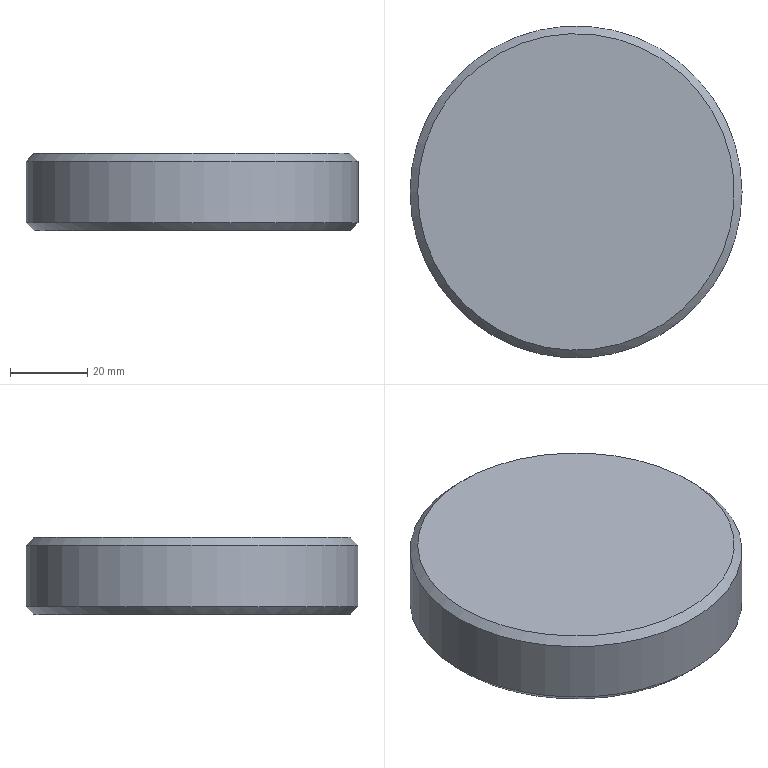Component | NX | CH3404_19_3-1 | 1 solid | 9 faces | box 86 x 86 x 20 mm | volume 33415 mm3 | plane 4 | cylinder 3 | cone 2 | commonest cylinder face diameters 86 x1 80 x1 82 x1
STEP:
#1=CARTESIAN_POINT('',(0.,0.,0.));
#2=DIRECTION('',(0.,0.,1.));
#3=DIRECTION('',(1.,0.,0.));
#4=AXIS2_PLACEMENT_3D('',#1,#2,#3);
#5=CARTESIAN_POINT('',(43.,0.,91.55));
#6=VERTEX_POINT('',#5);
#7=CARTESIAN_POINT('',(-43.,0.,91.55));
#8=VERTEX_POINT('',#7);
#9=CARTESIAN_POINT('',(-0.,0.,91.55));
#10=DIRECTION('',(0.,0.,1.));
#11=DIRECTION('',(1.,0.,0.));
#12=AXIS2_PLACEMENT_3D('',#9,#10,#11);
#13=CIRCLE('',#12,43.);
#14=CARTESIAN_POINT('',(-0.,0.,89.55));
#15=DIRECTION('',(0.,0.,-1.));
#16=DIRECTION('',(-1.,0.,0.));
#17=AXIS2_PLACEMENT_3D('',#14,#15,#16);
#18=CYLINDRICAL_SURFACE('',#17,43.);
#19=CARTESIAN_POINT('',(3.142,-2.));
#20=DIRECTION('',(-1.,0.));
#21=VECTOR('',#20,1.);
#22=LINE('',#19,#21);
#23=(GEOMETRIC_REPRESENTATION_CONTEXT(2)PARAMETRIC_REPRESENTATION_CONTEXT()REPRESENTATION_CONTEXT('',''));
#24=DEFINITIONAL_REPRESENTATION('',(#22),#23);
#25=PCURVE('',#18,#24);
#26=CARTESIAN_POINT('',(-0.,0.,89.55));
#27=DIRECTION('',(0.,0.,1.));
#28=DIRECTION('',(1.,0.,0.));
#29=AXIS2_PLACEMENT_3D('',#26,#27,#28);
#30=CONICAL_SURFACE('',#29,41.,0.7854);
#31=CARTESIAN_POINT('',(0.,2.));
#32=DIRECTION('',(1.,0.));
#33=VECTOR('',#32,1.);
#34=LINE('',#31,#33);
#35=(GEOMETRIC_REPRESENTATION_CONTEXT(2)PARAMETRIC_REPRESENTATION_CONTEXT()REPRESENTATION_CONTEXT('',''));
#36=DEFINITIONAL_REPRESENTATION('',(#34),#35);
#37=PCURVE('',#30,#36);
#38=SURFACE_CURVE('',#13,(#25,#37),.PCURVE_S1.);
#39=EDGE_CURVE('',#6,#8,#38,.T.);
#40=ORIENTED_EDGE('',*,*,#39,.T.);
#41=CARTESIAN_POINT('',(-43.,0.,107.55));
#42=VERTEX_POINT('',#41);
#43=CARTESIAN_POINT('',(-43.,-0.,107.55));
#44=CARTESIAN_POINT('',(-43.,-0.,91.55));
#45=B_SPLINE_CURVE_WITH_KNOTS('',1,(#43,#44),.UNSPECIFIED.,.F.,.F.,(2,2),(-18.,-2.),.PIECEWISE_BEZIER_KNOTS.);
#46=CARTESIAN_POINT('',(0.,0.));
#47=DIRECTION('',(0.,1.));
#48=VECTOR('',#47,1.);
#49=LINE('',#46,#48);
#50=(GEOMETRIC_REPRESENTATION_CONTEXT(2)PARAMETRIC_REPRESENTATION_CONTEXT()REPRESENTATION_CONTEXT('',''));
#51=DEFINITIONAL_REPRESENTATION('',(#49),#50);
#52=PCURVE('',#18,#51);
#53=CARTESIAN_POINT('',(6.283,0.));
#54=DIRECTION('',(0.,1.));
#55=VECTOR('',#54,1.);
#56=LINE('',#53,#55);
#57=(GEOMETRIC_REPRESENTATION_CONTEXT(2)PARAMETRIC_REPRESENTATION_CONTEXT()REPRESENTATION_CONTEXT('',''));
#58=DEFINITIONAL_REPRESENTATION('',(#56),#57);
#59=PCURVE('',#18,#58);
#60=SEAM_CURVE('',#45,(#52,#59),.PCURVE_S1.);
#61=EDGE_CURVE('',#42,#8,#60,.T.);
#62=ORIENTED_EDGE('',*,*,#61,.F.);
#63=CARTESIAN_POINT('',(-0.,0.,107.55));
#64=DIRECTION('',(0.,0.,-1.));
#65=DIRECTION('',(-1.,0.,0.));
#66=AXIS2_PLACEMENT_3D('',#63,#64,#65);
#67=CIRCLE('',#66,43.);
#68=CARTESIAN_POINT('',(0.,-18.));
#69=DIRECTION('',(1.,0.));
#70=VECTOR('',#69,1.);
#71=LINE('',#68,#70);
#72=(GEOMETRIC_REPRESENTATION_CONTEXT(2)PARAMETRIC_REPRESENTATION_CONTEXT()REPRESENTATION_CONTEXT('',''));
#73=DEFINITIONAL_REPRESENTATION('',(#71),#72);
#74=PCURVE('',#18,#73);
#75=CARTESIAN_POINT('',(-0.,0.,107.55));
#76=DIRECTION('',(0.,0.,-1.));
#77=DIRECTION('',(-1.,0.,0.));
#78=AXIS2_PLACEMENT_3D('',#75,#76,#77);
#79=CONICAL_SURFACE('',#78,43.,0.7854);
#80=CARTESIAN_POINT('',(0.,0.));
#81=DIRECTION('',(1.,0.));
#82=VECTOR('',#81,1.);
#83=LINE('',#80,#82);
#84=(GEOMETRIC_REPRESENTATION_CONTEXT(2)PARAMETRIC_REPRESENTATION_CONTEXT()REPRESENTATION_CONTEXT('',''));
#85=DEFINITIONAL_REPRESENTATION('',(#83),#84);
#86=PCURVE('',#79,#85);
#87=SURFACE_CURVE('',#67,(#74,#86),.PCURVE_S1.);
#88=EDGE_CURVE('',#42,#42,#87,.T.);
#89=ORIENTED_EDGE('',*,*,#88,.T.);
#90=ORIENTED_EDGE('',*,*,#61,.T.);
#91=CARTESIAN_POINT('',(-0.,0.,91.55));
#92=DIRECTION('',(0.,0.,1.));
#93=DIRECTION('',(1.,0.,0.));
#94=AXIS2_PLACEMENT_3D('',#91,#92,#93);
#95=CIRCLE('',#94,43.);
#96=CARTESIAN_POINT('',(9.425,-2.));
#97=DIRECTION('',(-1.,0.));
#98=VECTOR('',#97,1.);
#99=LINE('',#96,#98);
#100=(GEOMETRIC_REPRESENTATION_CONTEXT(2)PARAMETRIC_REPRESENTATION_CONTEXT()REPRESENTATION_CONTEXT('',''));
#101=DEFINITIONAL_REPRESENTATION('',(#99),#100);
#102=PCURVE('',#18,#101);
#103=CARTESIAN_POINT('',(0.,2.));
#104=DIRECTION('',(1.,0.));
#105=VECTOR('',#104,1.);
#106=LINE('',#103,#105);
#107=(GEOMETRIC_REPRESENTATION_CONTEXT(2)PARAMETRIC_REPRESENTATION_CONTEXT()REPRESENTATION_CONTEXT('',''));
#108=DEFINITIONAL_REPRESENTATION('',(#106),#107);
#109=PCURVE('',#30,#108);
#110=SURFACE_CURVE('',#95,(#102,#109),.PCURVE_S1.);
#111=EDGE_CURVE('',#8,#6,#110,.T.);
#112=ORIENTED_EDGE('',*,*,#111,.T.);
#113=EDGE_LOOP('',(#40,#62,#89,#90,#112));
#114=FACE_BOUND('',#113,.T.);
#115=ADVANCED_FACE('',(#114),#18,.T.);
#116=CARTESIAN_POINT('',(41.,0.,89.55));
#117=VERTEX_POINT('',#116);
#118=CARTESIAN_POINT('',(-0.,0.,89.55));
#119=DIRECTION('',(0.,0.,-1.));
#120=DIRECTION('',(1.,0.,0.));
#121=AXIS2_PLACEMENT_3D('',#118,#119,#120);
#122=CIRCLE('',#121,41.);
#123=CARTESIAN_POINT('',(-0.,-43.,89.55));
#124=DIRECTION('',(0.,0.,1.));
#125=DIRECTION('',(1.,0.,0.));
#126=AXIS2_PLACEMENT_3D('',#123,#124,#125);
#127=PLANE('',#126);
#128=CARTESIAN_POINT('',(41.,43.));
#129=CARTESIAN_POINT('',(41.,-28.014));
#130=CARTESIAN_POINT('',(-20.5,7.493));
#131=CARTESIAN_POINT('',(-82.,43.));
#132=CARTESIAN_POINT('',(-20.5,78.507));
#133=CARTESIAN_POINT('',(41.,114.014));
#134=CARTESIAN_POINT('',(41.,43.));
#135=(BOUNDED_CURVE()B_SPLINE_CURVE(2,(#128,#129,#130,#131,#132,#133,#134),.UNSPECIFIED.,.T.,.F.)B_SPLINE_CURVE_WITH_KNOTS((1,2,2,2,2,1),(-2.094,0.,2.094,4.189,6.283,8.378),.UNSPECIFIED.)CURVE()GEOMETRIC_REPRESENTATION_ITEM()RATIONAL_B_SPLINE_CURVE((1.,0.5,1.,0.5,1.,0.5,1.))REPRESENTATION_ITEM(''));
#136=(GEOMETRIC_REPRESENTATION_CONTEXT(2)PARAMETRIC_REPRESENTATION_CONTEXT()REPRESENTATION_CONTEXT('',''));
#137=DEFINITIONAL_REPRESENTATION('',(#135),#136);
#138=PCURVE('',#127,#137);
#139=CARTESIAN_POINT('',(6.283,0.));
#140=DIRECTION('',(-1.,0.));
#141=VECTOR('',#140,1.);
#142=LINE('',#139,#141);
#143=(GEOMETRIC_REPRESENTATION_CONTEXT(2)PARAMETRIC_REPRESENTATION_CONTEXT()REPRESENTATION_CONTEXT('',''));
#144=DEFINITIONAL_REPRESENTATION('',(#142),#143);
#145=PCURVE('',#30,#144);
#146=SURFACE_CURVE('',#122,(#138,#145),.PCURVE_S1.);
#147=EDGE_CURVE('',#117,#117,#146,.T.);
#148=ORIENTED_EDGE('',*,*,#147,.T.);
#149=EDGE_LOOP('',(#148));
#150=FACE_BOUND('',#149,.T.);
#151=CARTESIAN_POINT('',(-40.,0.,89.55));
#152=VERTEX_POINT('',#151);
#153=CARTESIAN_POINT('',(-0.,0.,89.55));
#154=DIRECTION('',(0.,0.,-1.));
#155=DIRECTION('',(-1.,0.,0.));
#156=AXIS2_PLACEMENT_3D('',#153,#154,#155);
#157=CIRCLE('',#156,40.);
#158=CARTESIAN_POINT('',(-40.,43.));
#159=CARTESIAN_POINT('',(-40.,112.282));
#160=CARTESIAN_POINT('',(20.,77.641));
#161=CARTESIAN_POINT('',(80.,43.));
#162=CARTESIAN_POINT('',(20.,8.359));
#163=CARTESIAN_POINT('',(-40.,-26.282));
#164=CARTESIAN_POINT('',(-40.,43.));
#165=(BOUNDED_CURVE()B_SPLINE_CURVE(2,(#158,#159,#160,#161,#162,#163,#164),.UNSPECIFIED.,.T.,.F.)B_SPLINE_CURVE_WITH_KNOTS((1,2,2,2,2,1),(-2.094,0.,2.094,4.189,6.283,8.378),.UNSPECIFIED.)CURVE()GEOMETRIC_REPRESENTATION_ITEM()RATIONAL_B_SPLINE_CURVE((1.,0.5,1.,0.5,1.,0.5,1.))REPRESENTATION_ITEM(''));
#166=(GEOMETRIC_REPRESENTATION_CONTEXT(2)PARAMETRIC_REPRESENTATION_CONTEXT()REPRESENTATION_CONTEXT('',''));
#167=DEFINITIONAL_REPRESENTATION('',(#165),#166);
#168=PCURVE('',#127,#167);
#169=CARTESIAN_POINT('',(-0.,0.,89.55));
#170=DIRECTION('',(0.,0.,-1.));
#171=DIRECTION('',(-1.,0.,0.));
#172=AXIS2_PLACEMENT_3D('',#169,#170,#171);
#173=CYLINDRICAL_SURFACE('',#172,40.);
#174=CARTESIAN_POINT('',(0.,0.));
#175=DIRECTION('',(1.,0.));
#176=VECTOR('',#175,1.);
#177=LINE('',#174,#176);
#178=(GEOMETRIC_REPRESENTATION_CONTEXT(2)PARAMETRIC_REPRESENTATION_CONTEXT()REPRESENTATION_CONTEXT('',''));
#179=DEFINITIONAL_REPRESENTATION('',(#177),#178);
#180=PCURVE('',#173,#179);
#181=SURFACE_CURVE('',#157,(#168,#180),.PCURVE_S1.);
#182=EDGE_CURVE('',#152,#152,#181,.T.);
#183=ORIENTED_EDGE('',*,*,#182,.F.);
#184=EDGE_LOOP('',(#183));
#185=FACE_BOUND('',#184,.T.);
#186=ADVANCED_FACE('',(#150,#185),#127,.F.);
#187=CARTESIAN_POINT('',(-40.,0.,100.55));
#188=VERTEX_POINT('',#187);
#189=CARTESIAN_POINT('',(-0.,0.,100.55));
#190=DIRECTION('',(0.,0.,-1.));
#191=DIRECTION('',(-1.,0.,0.));
#192=AXIS2_PLACEMENT_3D('',#189,#190,#191);
#193=CIRCLE('',#192,40.);
#194=CARTESIAN_POINT('',(0.,-11.));
#195=DIRECTION('',(1.,0.));
#196=VECTOR('',#195,1.);
#197=LINE('',#194,#196);
#198=(GEOMETRIC_REPRESENTATION_CONTEXT(2)PARAMETRIC_REPRESENTATION_CONTEXT()REPRESENTATION_CONTEXT('',''));
#199=DEFINITIONAL_REPRESENTATION('',(#197),#198);
#200=PCURVE('',#173,#199);
#201=CARTESIAN_POINT('',(-0.,-40.,100.55));
#202=DIRECTION('',(0.,0.,-1.));
#203=DIRECTION('',(-1.,0.,0.));
#204=AXIS2_PLACEMENT_3D('',#201,#202,#203);
#205=PLANE('',#204);
#206=CARTESIAN_POINT('',(0.,40.));
#207=DIRECTION('',(1.,0.));
#208=AXIS2_PLACEMENT_2D('',#206,#207);
#209=CIRCLE('',#208,40.);
#210=(GEOMETRIC_REPRESENTATION_CONTEXT(2)PARAMETRIC_REPRESENTATION_CONTEXT()REPRESENTATION_CONTEXT('',''));
#211=DEFINITIONAL_REPRESENTATION('',(#209),#210);
#212=PCURVE('',#205,#211);
#213=SURFACE_CURVE('',#193,(#200,#212),.PCURVE_S1.);
#214=EDGE_CURVE('',#188,#188,#213,.T.);
#215=ORIENTED_EDGE('',*,*,#214,.T.);
#216=CARTESIAN_POINT('',(-40.,0.,100.55));
#217=CARTESIAN_POINT('',(-40.,0.,89.55));
#218=B_SPLINE_CURVE_WITH_KNOTS('',1,(#216,#217),.UNSPECIFIED.,.F.,.F.,(2,2),(-11.,0.),.PIECEWISE_BEZIER_KNOTS.);
#219=CARTESIAN_POINT('',(6.283,0.));
#220=DIRECTION('',(0.,1.));
#221=VECTOR('',#220,1.);
#222=LINE('',#219,#221);
#223=(GEOMETRIC_REPRESENTATION_CONTEXT(2)PARAMETRIC_REPRESENTATION_CONTEXT()REPRESENTATION_CONTEXT('',''));
#224=DEFINITIONAL_REPRESENTATION('',(#222),#223);
#225=PCURVE('',#173,#224);
#226=CARTESIAN_POINT('',(0.,0.));
#227=DIRECTION('',(0.,1.));
#228=VECTOR('',#227,1.);
#229=LINE('',#226,#228);
#230=(GEOMETRIC_REPRESENTATION_CONTEXT(2)PARAMETRIC_REPRESENTATION_CONTEXT()REPRESENTATION_CONTEXT('',''));
#231=DEFINITIONAL_REPRESENTATION('',(#229),#230);
#232=PCURVE('',#173,#231);
#233=SEAM_CURVE('',#218,(#225,#232),.PCURVE_S1.);
#234=EDGE_CURVE('',#188,#152,#233,.T.);
#235=ORIENTED_EDGE('',*,*,#234,.T.);
#236=ORIENTED_EDGE('',*,*,#182,.F.);
#237=ORIENTED_EDGE('',*,*,#234,.F.);
#238=EDGE_LOOP('',(#215,#235,#236,#237));
#239=FACE_BOUND('',#238,.F.);
#240=ADVANCED_FACE('',(#239),#173,.F.);
#241=CARTESIAN_POINT('',(-41.,0.,100.55));
#242=VERTEX_POINT('',#241);
#243=CARTESIAN_POINT('',(-0.,0.,100.55));
#244=DIRECTION('',(0.,0.,-1.));
#245=DIRECTION('',(-1.,0.,0.));
#246=AXIS2_PLACEMENT_3D('',#243,#244,#245);
#247=CIRCLE('',#246,41.);
#248=CARTESIAN_POINT('',(0.,40.));
#249=DIRECTION('',(1.,0.));
#250=AXIS2_PLACEMENT_2D('',#248,#249);
#251=CIRCLE('',#250,41.);
#252=(GEOMETRIC_REPRESENTATION_CONTEXT(2)PARAMETRIC_REPRESENTATION_CONTEXT()REPRESENTATION_CONTEXT('',''));
#253=DEFINITIONAL_REPRESENTATION('',(#251),#252);
#254=PCURVE('',#205,#253);
#255=CARTESIAN_POINT('',(-0.,0.,89.55));
#256=DIRECTION('',(0.,0.,-1.));
#257=DIRECTION('',(-1.,0.,0.));
#258=AXIS2_PLACEMENT_3D('',#255,#256,#257);
#259=CYLINDRICAL_SURFACE('',#258,41.);
#260=CARTESIAN_POINT('',(0.,-11.));
#261=DIRECTION('',(1.,0.));
#262=VECTOR('',#261,1.);
#263=LINE('',#260,#262);
#264=(GEOMETRIC_REPRESENTATION_CONTEXT(2)PARAMETRIC_REPRESENTATION_CONTEXT()REPRESENTATION_CONTEXT('',''));
#265=DEFINITIONAL_REPRESENTATION('',(#263),#264);
#266=PCURVE('',#259,#265);
#267=SURFACE_CURVE('',#247,(#254,#266),.PCURVE_S1.);
#268=EDGE_CURVE('',#242,#242,#267,.T.);
#269=ORIENTED_EDGE('',*,*,#268,.F.);
#270=EDGE_LOOP('',(#269));
#271=FACE_BOUND('',#270,.T.);
#272=ORIENTED_EDGE('',*,*,#214,.T.);
#273=EDGE_LOOP('',(#272));
#274=FACE_BOUND('',#273,.T.);
#275=ADVANCED_FACE('',(#271,#274),#205,.F.);
#276=CARTESIAN_POINT('',(-41.,0.,105.55));
#277=VERTEX_POINT('',#276);
#278=CARTESIAN_POINT('',(-0.,0.,105.55));
#279=DIRECTION('',(0.,0.,-1.));
#280=DIRECTION('',(-1.,0.,0.));
#281=AXIS2_PLACEMENT_3D('',#278,#279,#280);
#282=CIRCLE('',#281,41.);
#283=CARTESIAN_POINT('',(0.,-16.));
#284=DIRECTION('',(1.,0.));
#285=VECTOR('',#284,1.);
#286=LINE('',#283,#285);
#287=(GEOMETRIC_REPRESENTATION_CONTEXT(2)PARAMETRIC_REPRESENTATION_CONTEXT()REPRESENTATION_CONTEXT('',''));
#288=DEFINITIONAL_REPRESENTATION('',(#286),#287);
#289=PCURVE('',#259,#288);
#290=CARTESIAN_POINT('',(-0.,-41.,105.55));
#291=DIRECTION('',(0.,0.,1.));
#292=DIRECTION('',(1.,0.,0.));
#293=AXIS2_PLACEMENT_3D('',#290,#291,#292);
#294=PLANE('',#293);
#295=CARTESIAN_POINT('',(-41.,41.));
#296=CARTESIAN_POINT('',(-41.,112.014));
#297=CARTESIAN_POINT('',(20.5,76.507));
#298=CARTESIAN_POINT('',(82.,41.));
#299=CARTESIAN_POINT('',(20.5,5.493));
#300=CARTESIAN_POINT('',(-41.,-30.014));
#301=CARTESIAN_POINT('',(-41.,41.));
#302=(BOUNDED_CURVE()B_SPLINE_CURVE(2,(#295,#296,#297,#298,#299,#300,#301),.UNSPECIFIED.,.T.,.F.)B_SPLINE_CURVE_WITH_KNOTS((1,2,2,2,2,1),(-2.094,0.,2.094,4.189,6.283,8.378),.UNSPECIFIED.)CURVE()GEOMETRIC_REPRESENTATION_ITEM()RATIONAL_B_SPLINE_CURVE((1.,0.5,1.,0.5,1.,0.5,1.))REPRESENTATION_ITEM(''));
#303=(GEOMETRIC_REPRESENTATION_CONTEXT(2)PARAMETRIC_REPRESENTATION_CONTEXT()REPRESENTATION_CONTEXT('',''));
#304=DEFINITIONAL_REPRESENTATION('',(#302),#303);
#305=PCURVE('',#294,#304);
#306=SURFACE_CURVE('',#282,(#289,#305),.PCURVE_S1.);
#307=EDGE_CURVE('',#277,#277,#306,.T.);
#308=ORIENTED_EDGE('',*,*,#307,.T.);
#309=CARTESIAN_POINT('',(-41.,0.,105.55));
#310=CARTESIAN_POINT('',(-41.,0.,100.55));
#311=B_SPLINE_CURVE_WITH_KNOTS('',1,(#309,#310),.UNSPECIFIED.,.F.,.F.,(2,2),(-16.,-11.),.PIECEWISE_BEZIER_KNOTS.);
#312=CARTESIAN_POINT('',(6.283,0.));
#313=DIRECTION('',(0.,1.));
#314=VECTOR('',#313,1.);
#315=LINE('',#312,#314);
#316=(GEOMETRIC_REPRESENTATION_CONTEXT(2)PARAMETRIC_REPRESENTATION_CONTEXT()REPRESENTATION_CONTEXT('',''));
#317=DEFINITIONAL_REPRESENTATION('',(#315),#316);
#318=PCURVE('',#259,#317);
#319=CARTESIAN_POINT('',(0.,0.));
#320=DIRECTION('',(0.,1.));
#321=VECTOR('',#320,1.);
#322=LINE('',#319,#321);
#323=(GEOMETRIC_REPRESENTATION_CONTEXT(2)PARAMETRIC_REPRESENTATION_CONTEXT()REPRESENTATION_CONTEXT('',''));
#324=DEFINITIONAL_REPRESENTATION('',(#322),#323);
#325=PCURVE('',#259,#324);
#326=SEAM_CURVE('',#311,(#318,#325),.PCURVE_S1.);
#327=EDGE_CURVE('',#277,#242,#326,.T.);
#328=ORIENTED_EDGE('',*,*,#327,.T.);
#329=ORIENTED_EDGE('',*,*,#268,.F.);
#330=ORIENTED_EDGE('',*,*,#327,.F.);
#331=EDGE_LOOP('',(#308,#328,#329,#330));
#332=FACE_BOUND('',#331,.F.);
#333=ADVANCED_FACE('',(#332),#259,.F.);
#334=ORIENTED_EDGE('',*,*,#307,.T.);
#335=EDGE_LOOP('',(#334));
#336=FACE_BOUND('',#335,.T.);
#337=ADVANCED_FACE('',(#336),#294,.F.);
#338=CARTESIAN_POINT('',(-41.,0.,109.55));
#339=VERTEX_POINT('',#338);
#340=CARTESIAN_POINT('',(-0.,0.,109.55));
#341=DIRECTION('',(0.,0.,1.));
#342=DIRECTION('',(-1.,0.,0.));
#343=AXIS2_PLACEMENT_3D('',#340,#341,#342);
#344=CIRCLE('',#343,41.);
#345=CARTESIAN_POINT('',(-0.,0.,109.55));
#346=DIRECTION('',(0.,0.,-1.));
#347=DIRECTION('',(-1.,0.,0.));
#348=AXIS2_PLACEMENT_3D('',#345,#346,#347);
#349=PLANE('',#348);
#350=CARTESIAN_POINT('',(41.,0.));
#351=CARTESIAN_POINT('',(41.,-71.014));
#352=CARTESIAN_POINT('',(-20.5,-35.507));
#353=CARTESIAN_POINT('',(-82.,-0.));
#354=CARTESIAN_POINT('',(-20.5,35.507));
#355=CARTESIAN_POINT('',(41.,71.014));
#356=CARTESIAN_POINT('',(41.,0.));
#357=(BOUNDED_CURVE()B_SPLINE_CURVE(2,(#350,#351,#352,#353,#354,#355,#356),.UNSPECIFIED.,.T.,.F.)B_SPLINE_CURVE_WITH_KNOTS((1,2,2,2,2,1),(-2.094,0.,2.094,4.189,6.283,8.378),.UNSPECIFIED.)CURVE()GEOMETRIC_REPRESENTATION_ITEM()RATIONAL_B_SPLINE_CURVE((1.,0.5,1.,0.5,1.,0.5,1.))REPRESENTATION_ITEM(''));
#358=(GEOMETRIC_REPRESENTATION_CONTEXT(2)PARAMETRIC_REPRESENTATION_CONTEXT()REPRESENTATION_CONTEXT('',''));
#359=DEFINITIONAL_REPRESENTATION('',(#357),#358);
#360=PCURVE('',#349,#359);
#361=CARTESIAN_POINT('',(6.283,-2.));
#362=DIRECTION('',(-1.,0.));
#363=VECTOR('',#362,1.);
#364=LINE('',#361,#363);
#365=(GEOMETRIC_REPRESENTATION_CONTEXT(2)PARAMETRIC_REPRESENTATION_CONTEXT()REPRESENTATION_CONTEXT('',''));
#366=DEFINITIONAL_REPRESENTATION('',(#364),#365);
#367=PCURVE('',#79,#366);
#368=SURFACE_CURVE('',#344,(#360,#367),.PCURVE_S1.);
#369=EDGE_CURVE('',#339,#339,#368,.T.);
#370=ORIENTED_EDGE('',*,*,#369,.T.);
#371=EDGE_LOOP('',(#370));
#372=FACE_BOUND('',#371,.T.);
#373=ADVANCED_FACE('',(#372),#349,.F.);
#374=ORIENTED_EDGE('',*,*,#39,.F.);
#375=CARTESIAN_POINT('',(41.,-0.,89.55));
#376=CARTESIAN_POINT('',(43.,-0.,91.55));
#377=B_SPLINE_CURVE_WITH_KNOTS('',1,(#375,#376),.UNSPECIFIED.,.F.,.F.,(2,2),(0.,2.828),.PIECEWISE_BEZIER_KNOTS.);
#378=CARTESIAN_POINT('',(0.,0.));
#379=DIRECTION('',(0.,1.));
#380=VECTOR('',#379,1.);
#381=LINE('',#378,#380);
#382=(GEOMETRIC_REPRESENTATION_CONTEXT(2)PARAMETRIC_REPRESENTATION_CONTEXT()REPRESENTATION_CONTEXT('',''));
#383=DEFINITIONAL_REPRESENTATION('',(#381),#382);
#384=PCURVE('',#30,#383);
#385=CARTESIAN_POINT('',(6.283,0.));
#386=DIRECTION('',(0.,1.));
#387=VECTOR('',#386,1.);
#388=LINE('',#385,#387);
#389=(GEOMETRIC_REPRESENTATION_CONTEXT(2)PARAMETRIC_REPRESENTATION_CONTEXT()REPRESENTATION_CONTEXT('',''));
#390=DEFINITIONAL_REPRESENTATION('',(#388),#389);
#391=PCURVE('',#30,#390);
#392=SEAM_CURVE('',#377,(#384,#391),.PCURVE_S1.);
#393=EDGE_CURVE('',#117,#6,#392,.T.);
#394=ORIENTED_EDGE('',*,*,#393,.F.);
#395=ORIENTED_EDGE('',*,*,#147,.F.);
#396=ORIENTED_EDGE('',*,*,#393,.T.);
#397=ORIENTED_EDGE('',*,*,#111,.F.);
#398=EDGE_LOOP('',(#374,#394,#395,#396,#397));
#399=FACE_BOUND('',#398,.T.);
#400=ADVANCED_FACE('',(#399),#30,.T.);
#401=ORIENTED_EDGE('',*,*,#369,.F.);
#402=CARTESIAN_POINT('',(-41.,0.,109.55));
#403=CARTESIAN_POINT('',(-43.,0.,107.55));
#404=B_SPLINE_CURVE_WITH_KNOTS('',1,(#402,#403),.UNSPECIFIED.,.F.,.F.,(2,2),(-2.828,0.),.PIECEWISE_BEZIER_KNOTS.);
#405=CARTESIAN_POINT('',(6.283,0.));
#406=DIRECTION('',(0.,1.));
#407=VECTOR('',#406,1.);
#408=LINE('',#405,#407);
#409=(GEOMETRIC_REPRESENTATION_CONTEXT(2)PARAMETRIC_REPRESENTATION_CONTEXT()REPRESENTATION_CONTEXT('',''));
#410=DEFINITIONAL_REPRESENTATION('',(#408),#409);
#411=PCURVE('',#79,#410);
#412=CARTESIAN_POINT('',(0.,0.));
#413=DIRECTION('',(0.,1.));
#414=VECTOR('',#413,1.);
#415=LINE('',#412,#414);
#416=(GEOMETRIC_REPRESENTATION_CONTEXT(2)PARAMETRIC_REPRESENTATION_CONTEXT()REPRESENTATION_CONTEXT('',''));
#417=DEFINITIONAL_REPRESENTATION('',(#415),#416);
#418=PCURVE('',#79,#417);
#419=SEAM_CURVE('',#404,(#411,#418),.PCURVE_S1.);
#420=EDGE_CURVE('',#339,#42,#419,.T.);
#421=ORIENTED_EDGE('',*,*,#420,.T.);
#422=ORIENTED_EDGE('',*,*,#88,.F.);
#423=ORIENTED_EDGE('',*,*,#420,.F.);
#424=EDGE_LOOP('',(#401,#421,#422,#423));
#425=FACE_BOUND('',#424,.T.);
#426=ADVANCED_FACE('',(#425),#79,.T.);
#427=CLOSED_SHELL('',(#115,#186,#240,#275,#333,#337,#373,#400,#426));
#428=MANIFOLD_SOLID_BREP('',#427);
#429=(LENGTH_UNIT()NAMED_UNIT(*)SI_UNIT(.MILLI.,.METRE.));
#430=UNCERTAINTY_MEASURE_WITH_UNIT(LENGTH_MEASURE(0.00001),#429,'','');
#431=(NAMED_UNIT(*)PLANE_ANGLE_UNIT()SI_UNIT($,.RADIAN.));
#432=(NAMED_UNIT(*)SI_UNIT($,.STERADIAN.)SOLID_ANGLE_UNIT());
#433=(GEOMETRIC_REPRESENTATION_CONTEXT(3)GLOBAL_UNCERTAINTY_ASSIGNED_CONTEXT((#430))GLOBAL_UNIT_ASSIGNED_CONTEXT((#429,#431,#432))REPRESENTATION_CONTEXT('',''));
#434=ADVANCED_BREP_SHAPE_REPRESENTATION('',(#4,#428),#433);